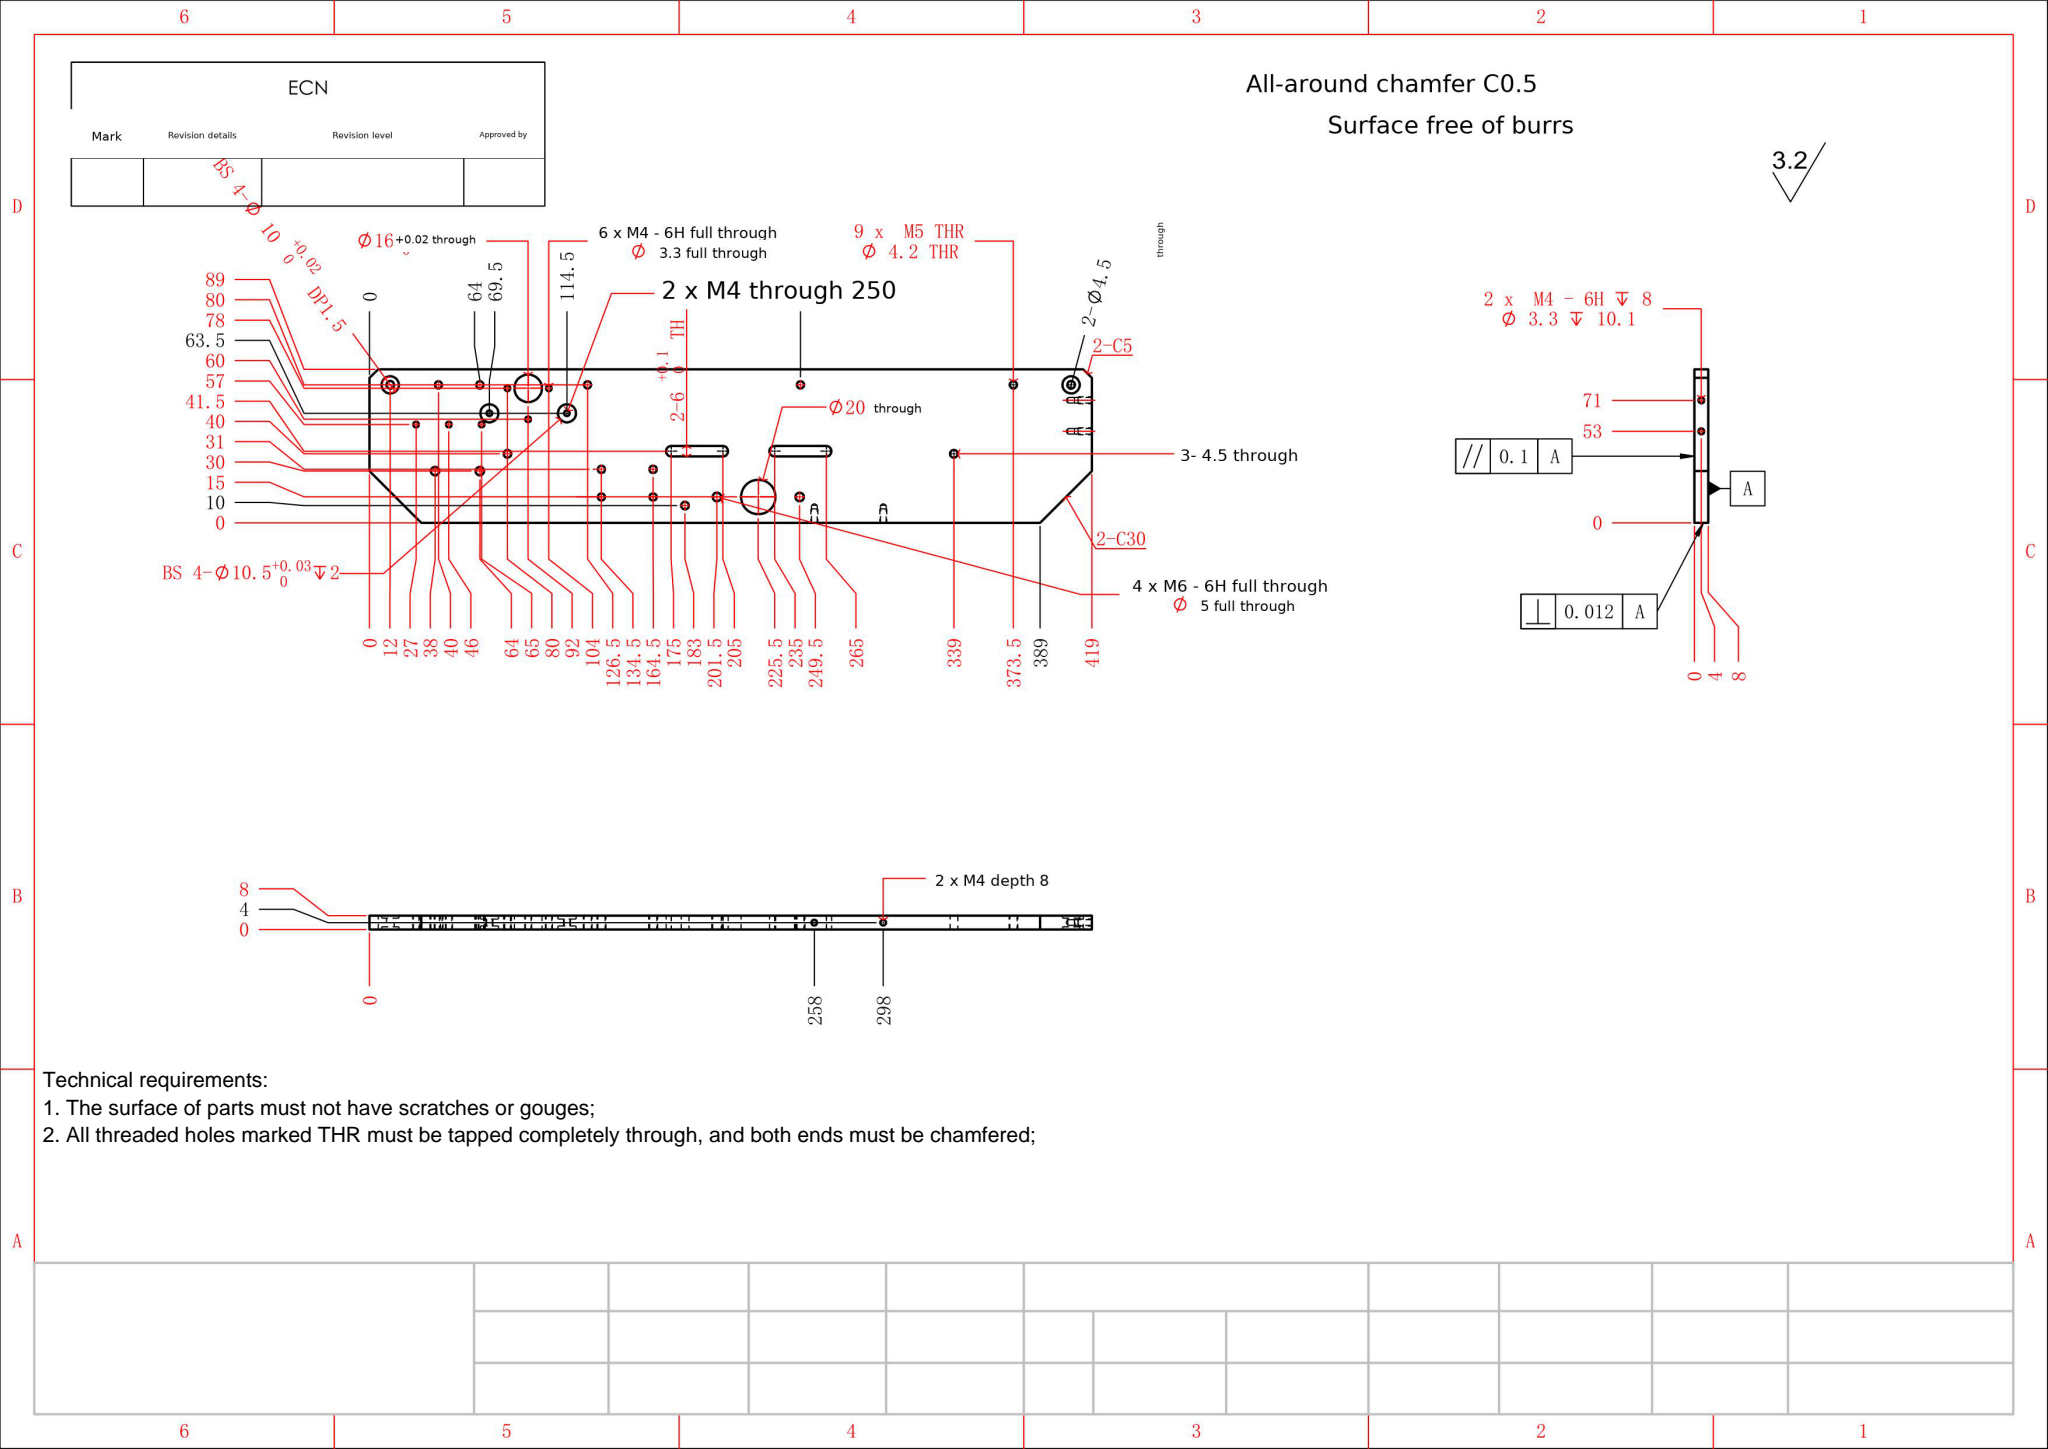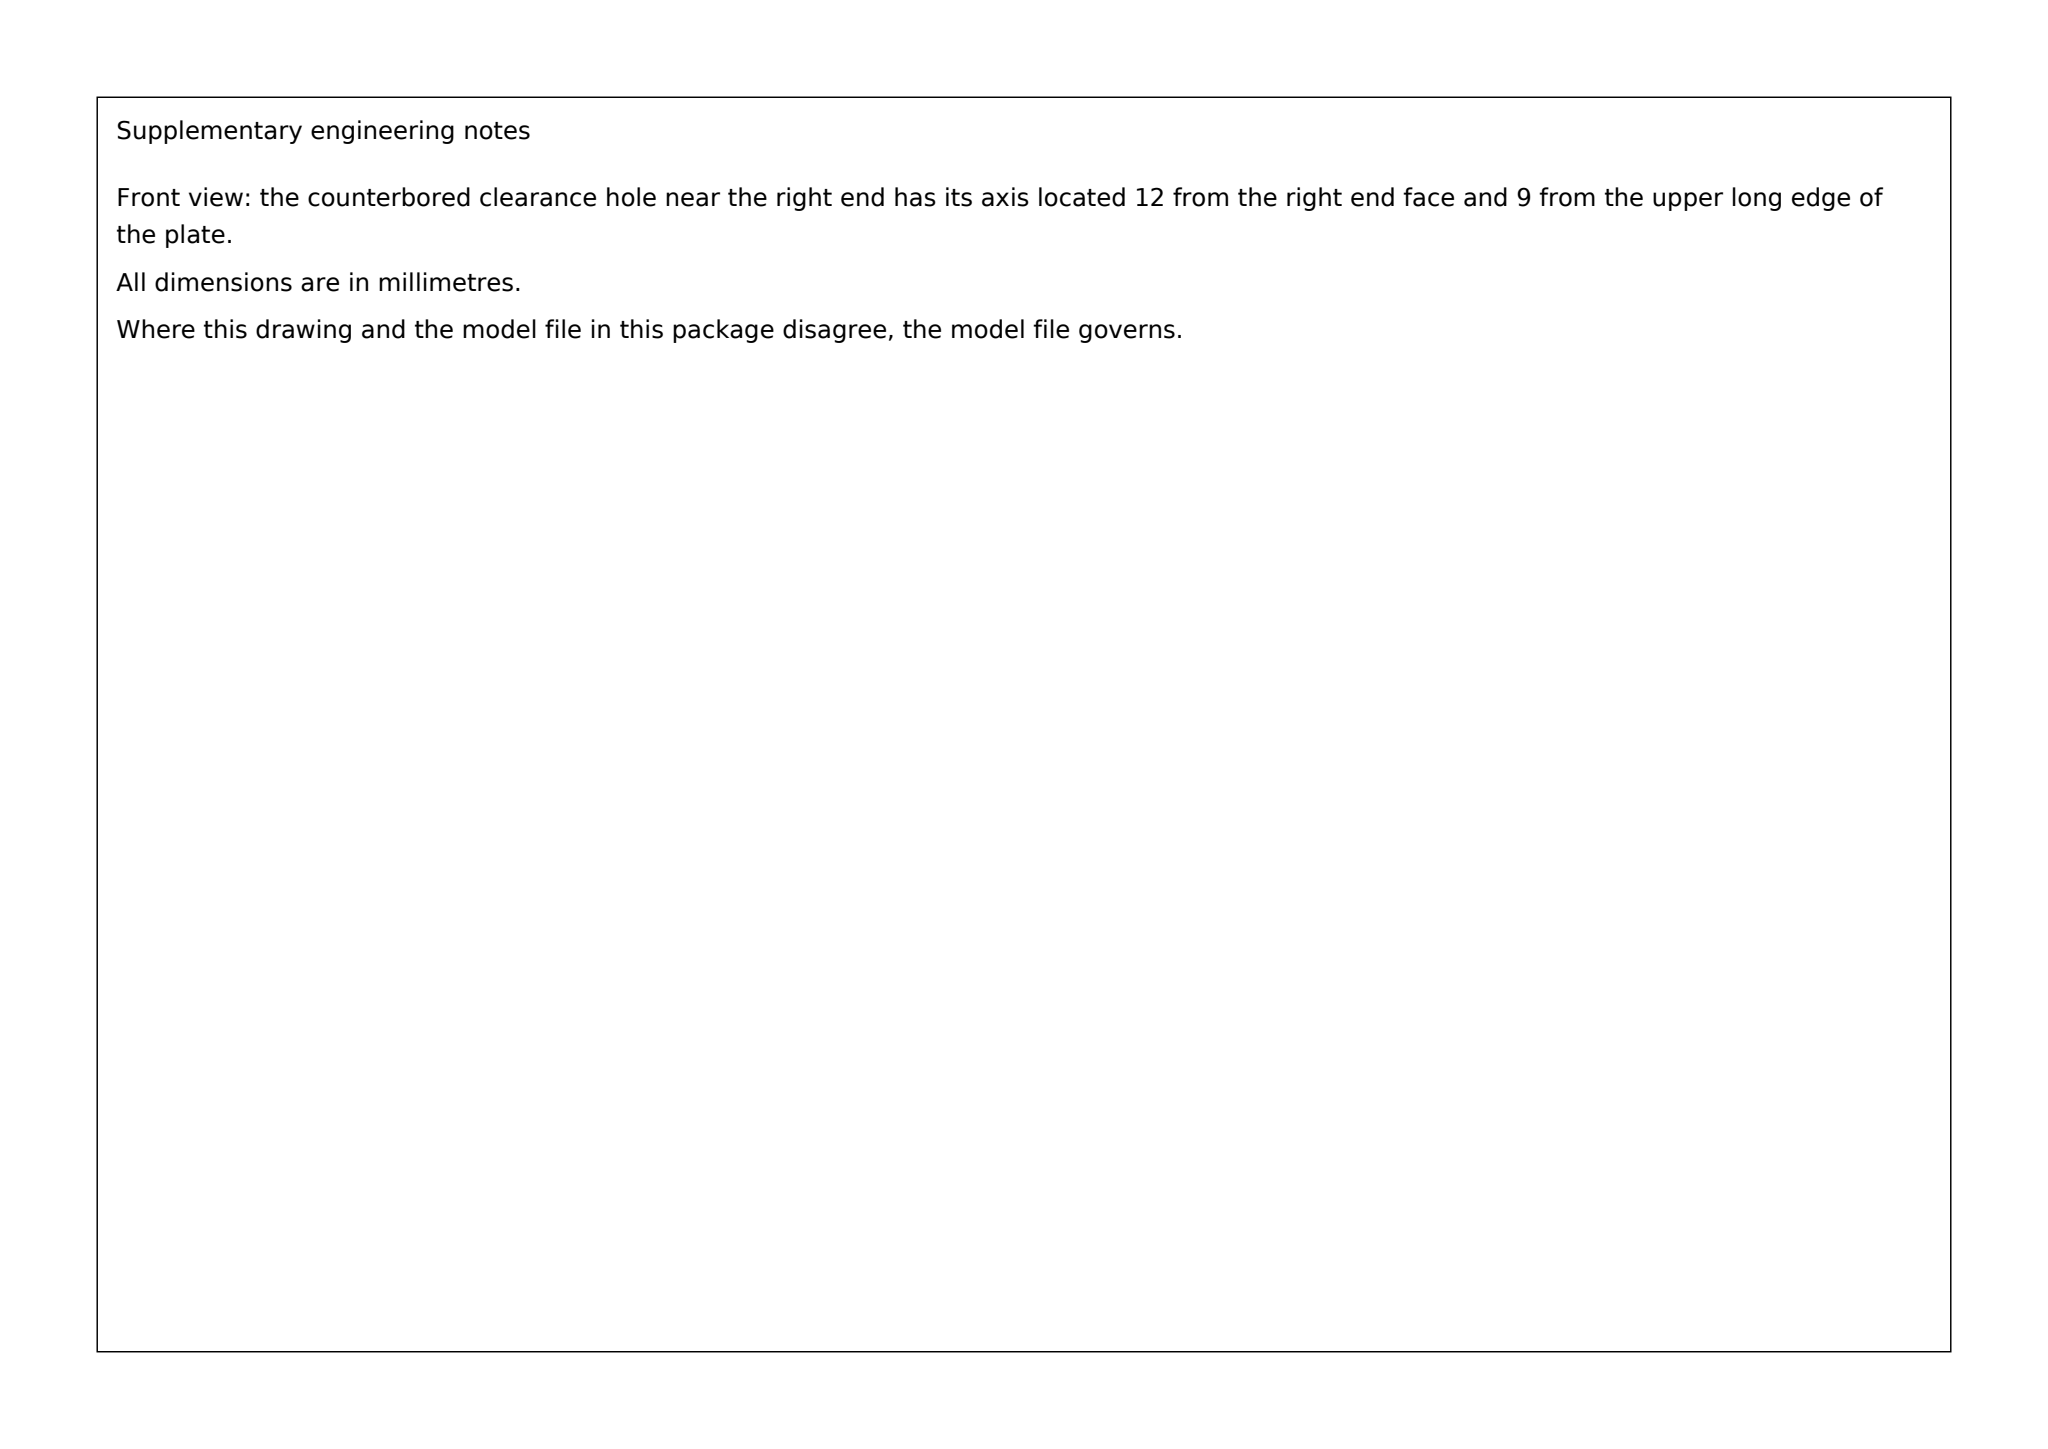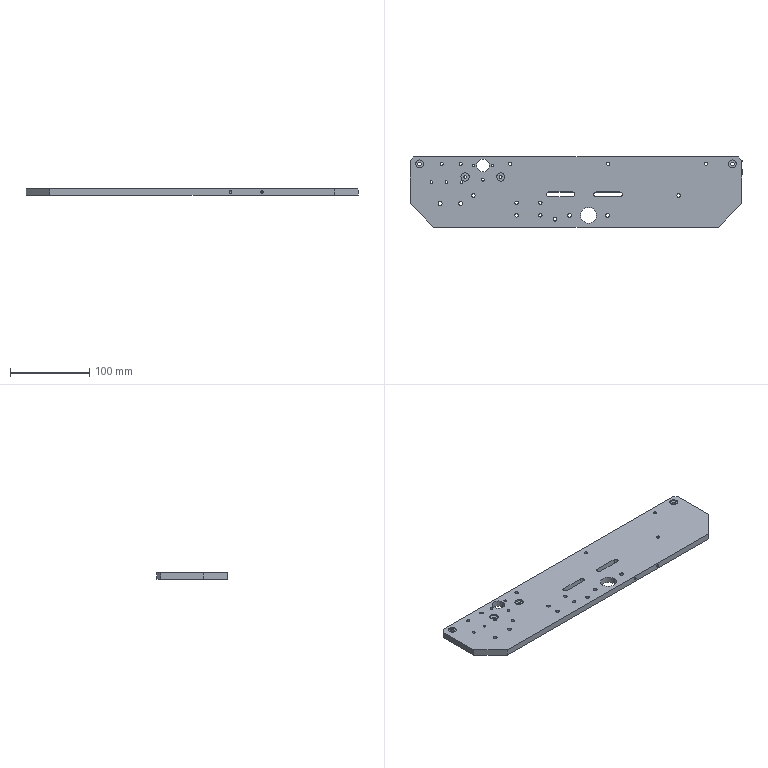Part | SolidWorks | mm | 1 solid | 124 faces | box 419 x 89 x 8 mm | volume 279243 mm3 | cylinder 90 | plane 22 | cone 12 | commonest cylinder face diameters 3.3 x24 4.2 x18 4.5 x10 10.5 x8 10 x8 5 x8 6 x6 3.242 x4
Drawing notes:
OVERALL PLATE 419 x 89 x 8 | from the solid: bbox_xyz [419.0, 89.0, 8.0]
3X Ø4.5 THRU: X80 Y40, X183 Y10, X339 Y40 | from the solid: Ø4.5 z-cyls len 8 at [80,40],[183,10],[339,40]
2X Ø4.5 THRU, CBORE Ø10 DP1.5, AT X12 & X407, Y80 | from the solid: Ø4.5 z-cyl len 5 + Ø10 z-cyl len 1.5 at [12,80] and [407,80]
2X Ø3.3 DP4, CBORE Ø10.5 +0.03/0 DP2, AT X69.5 & X114.5, Y63.5 | from the solid: Ø3.3 z-cyl len 4 at [69.5,63.5] & [114.5,63.5]; Ø10.5 z-cyl len 2 same positions
2X SLOT W6 x 36 OAL, R3 ENDS, THRU; CL Y41.5, X175/205 & X235/265 | from the solid: Ø6 thru cyls len 8 at [175,41.5],[205,41.5] and [235,41.5],[265,41.5]; 30 c-c + Ø6 = 36 OAL
2X M4-6H DP8, Ø3.3 DP10.1 IN LONG EDGE AT X258 & X298, Z4 | from the solid: Ø3.3 y-axis cyls len 10.1 at [258,-,4] and [298,-,4]
M5 THR (Ø4.2 THR): X250 FROM LH EDGE, Y80 FROM BTM EDGE | from the solid: cylinder dia 4.2 axis z at pos [250.0, 80.0], length 8.0 (full thru 8 thk)